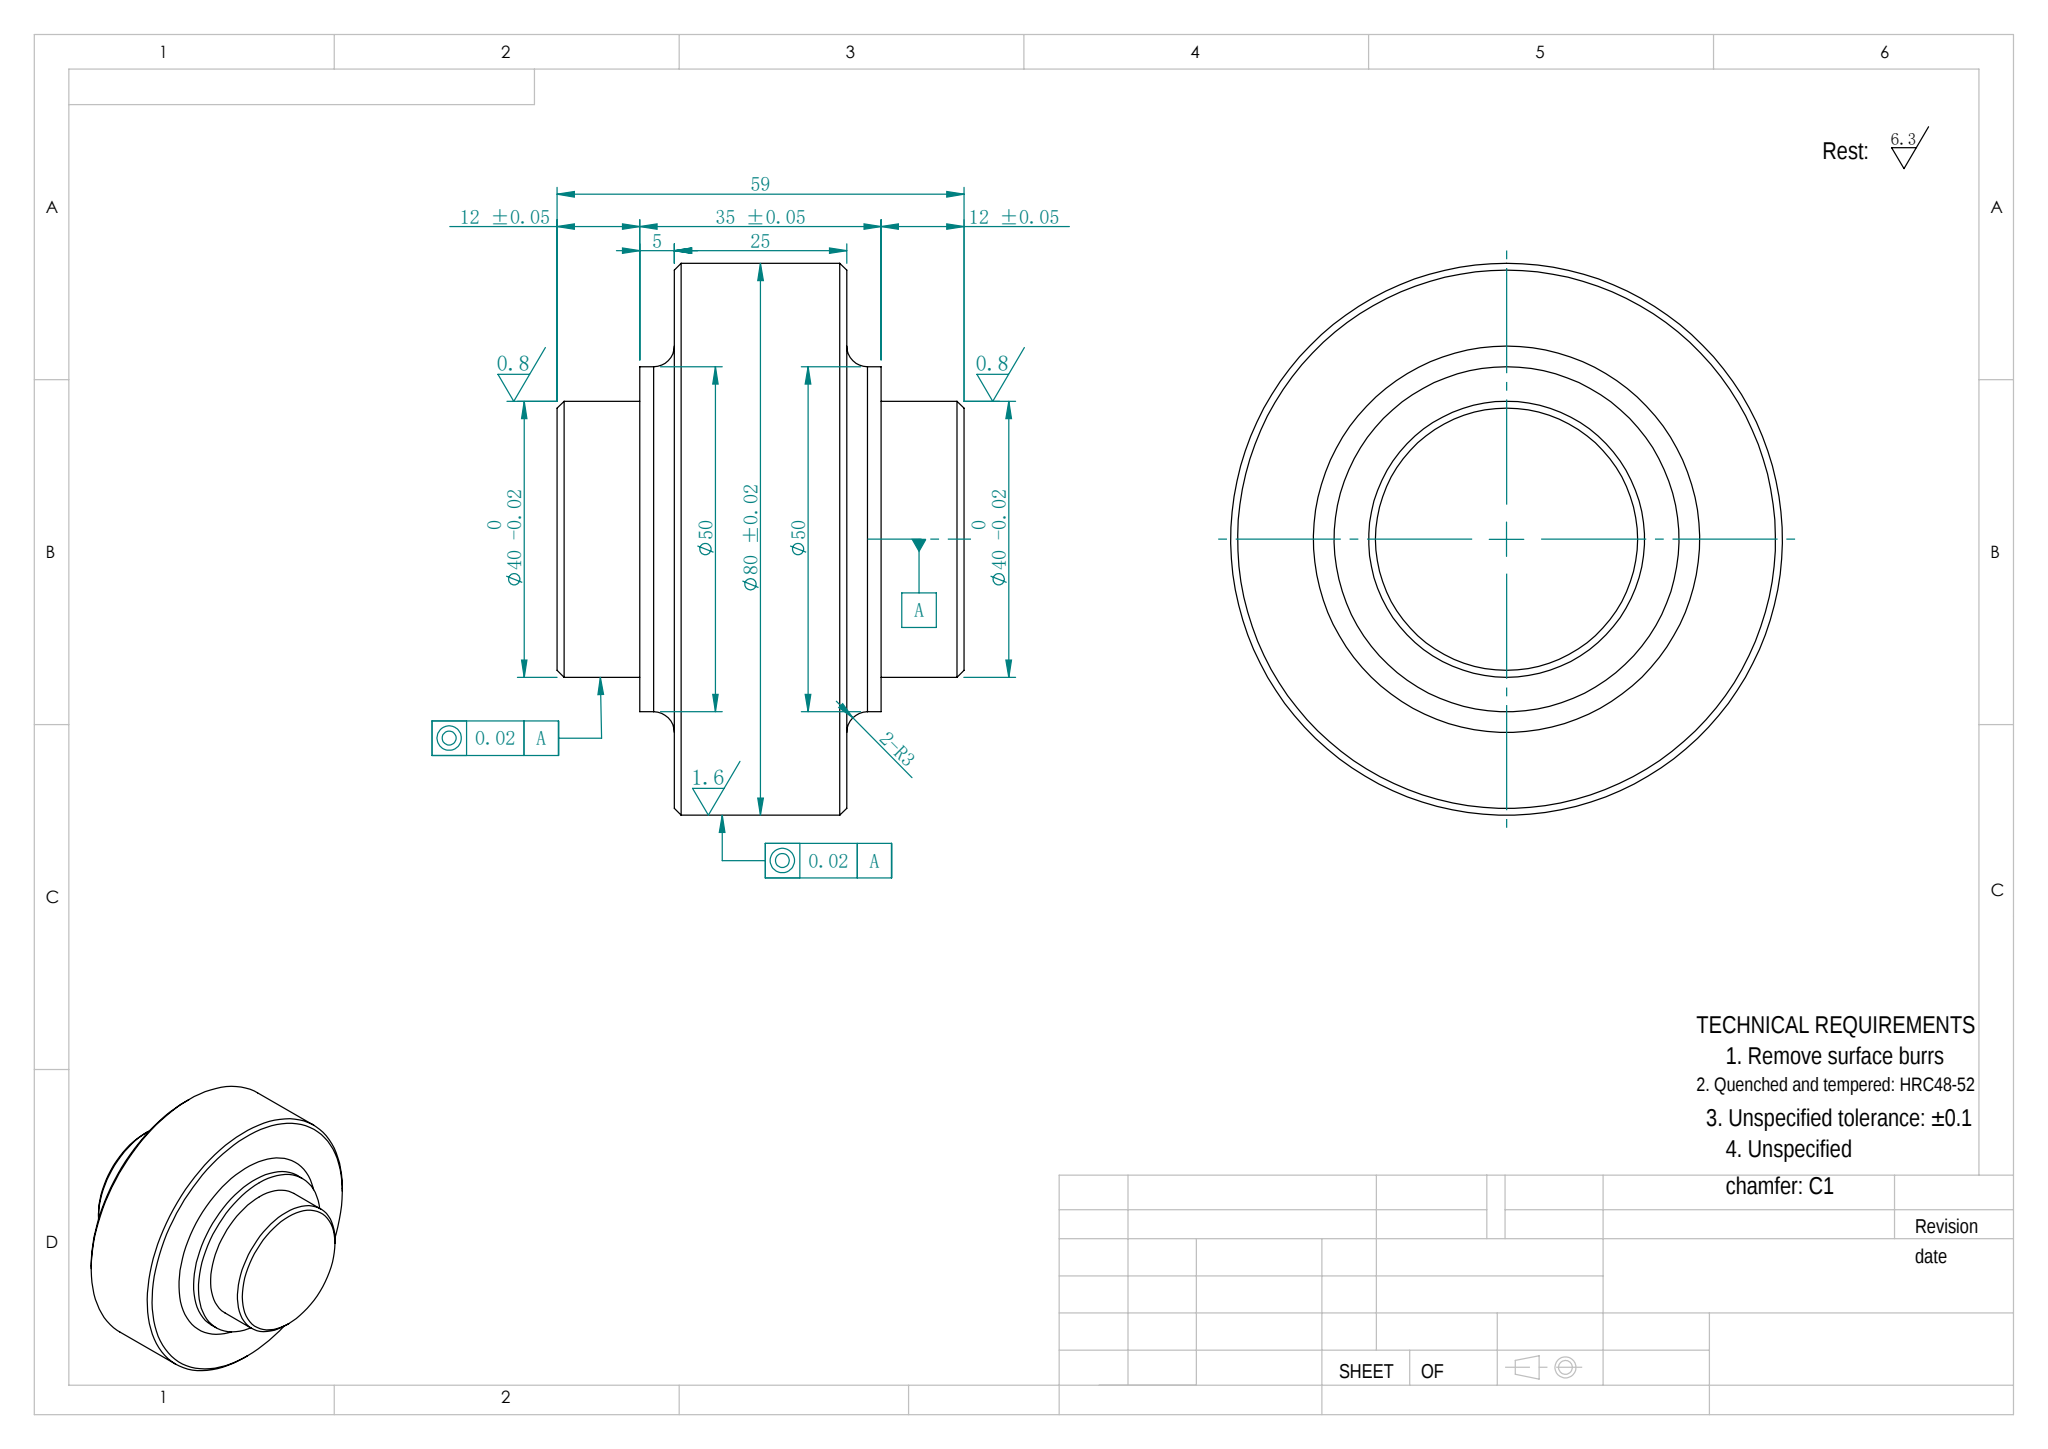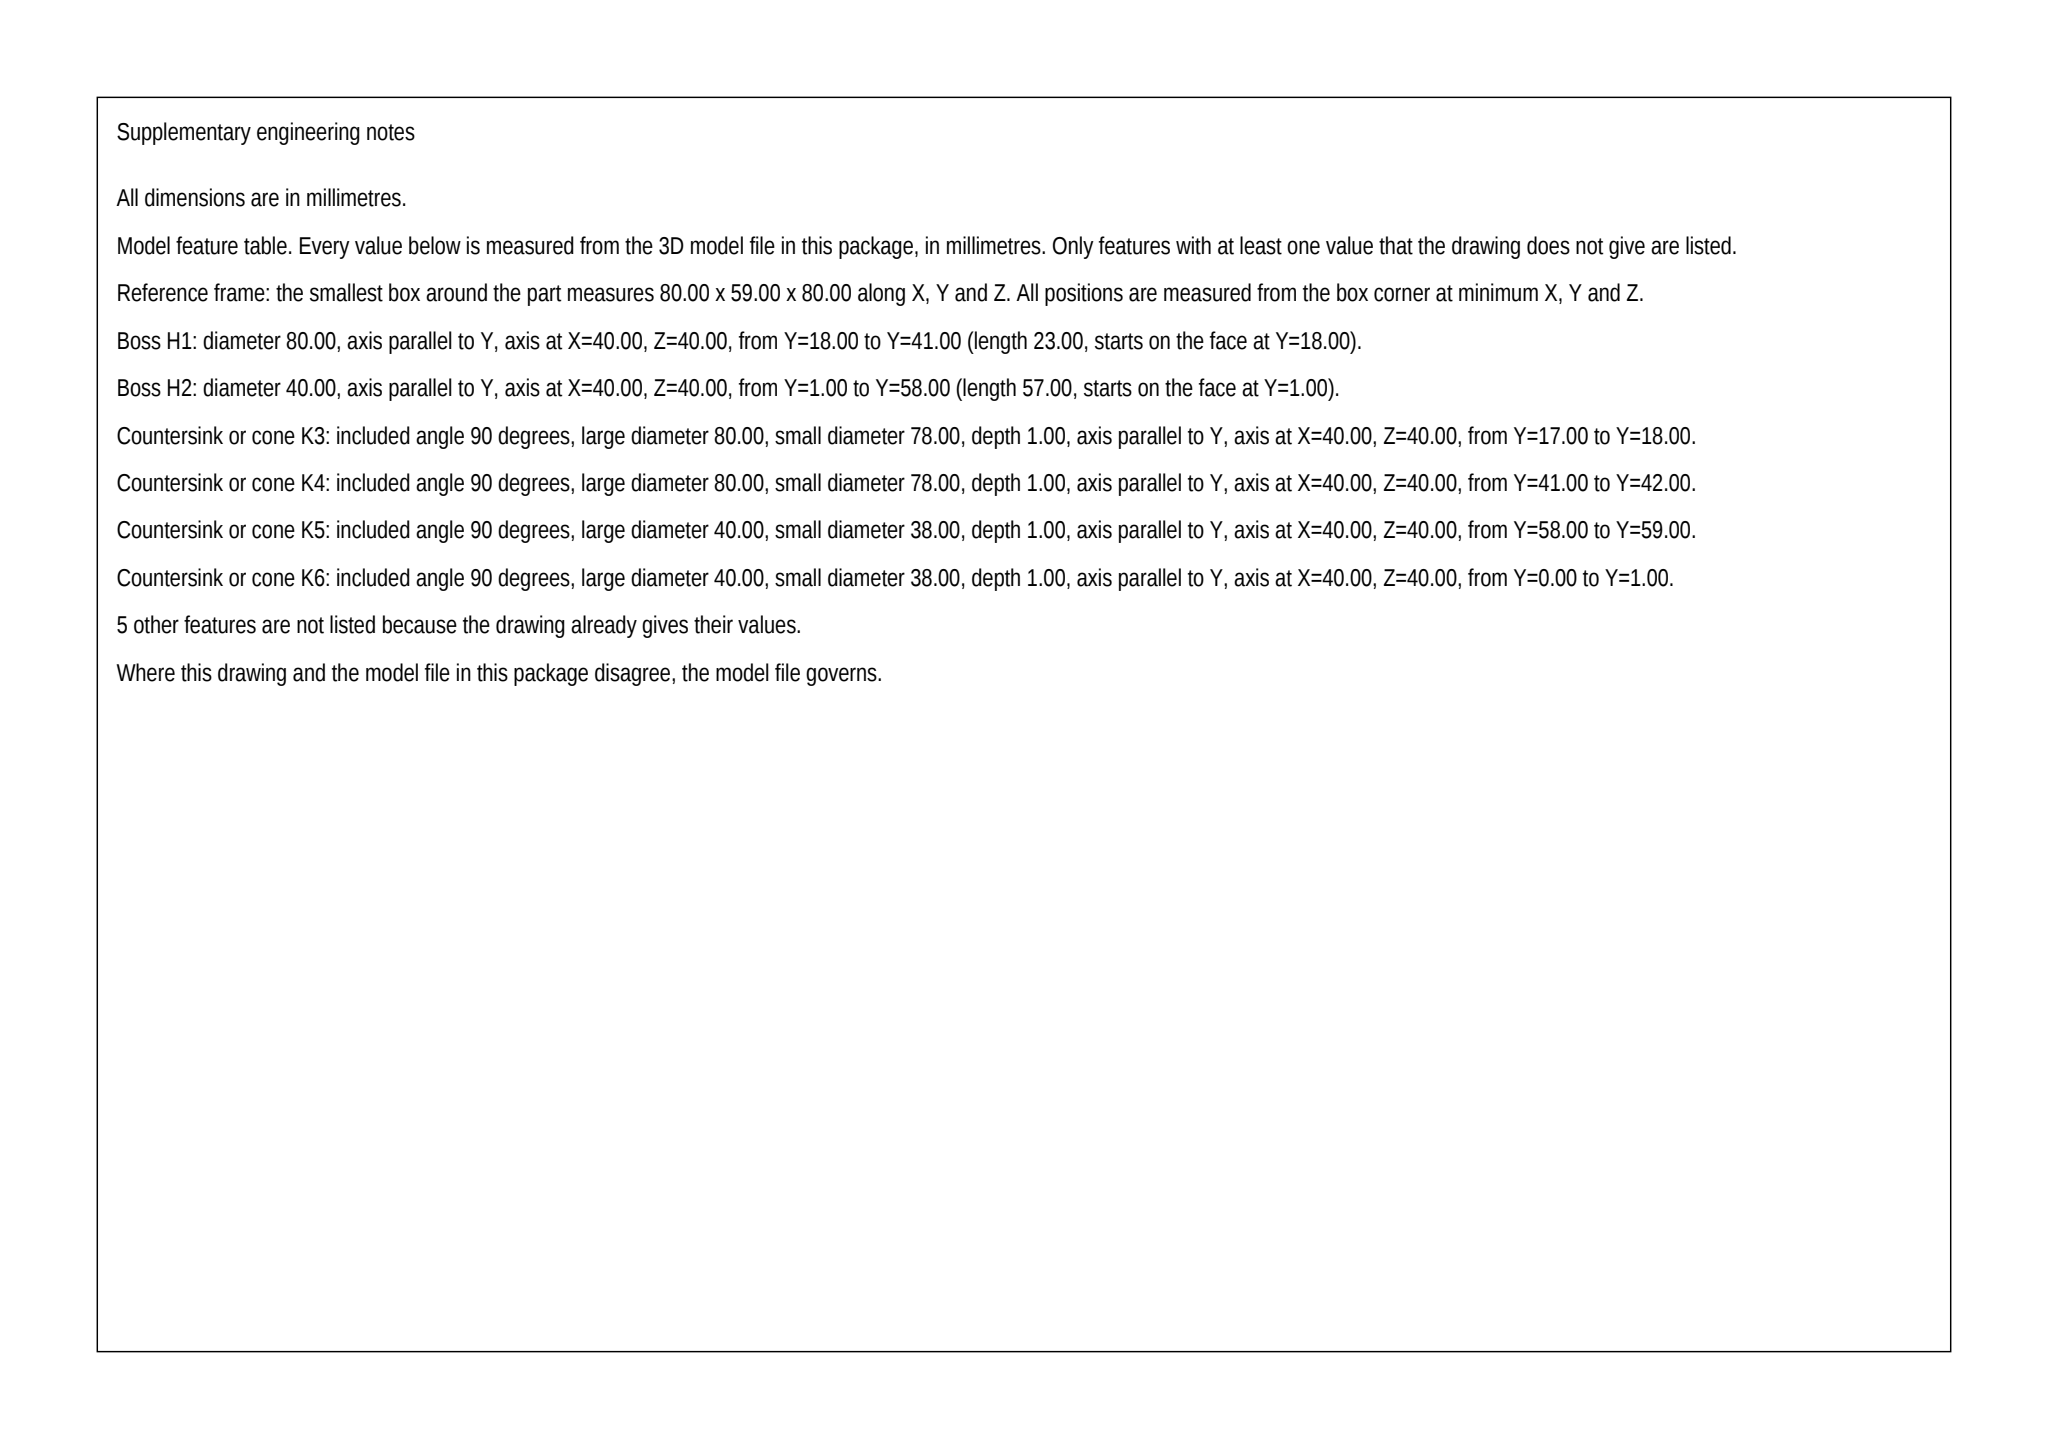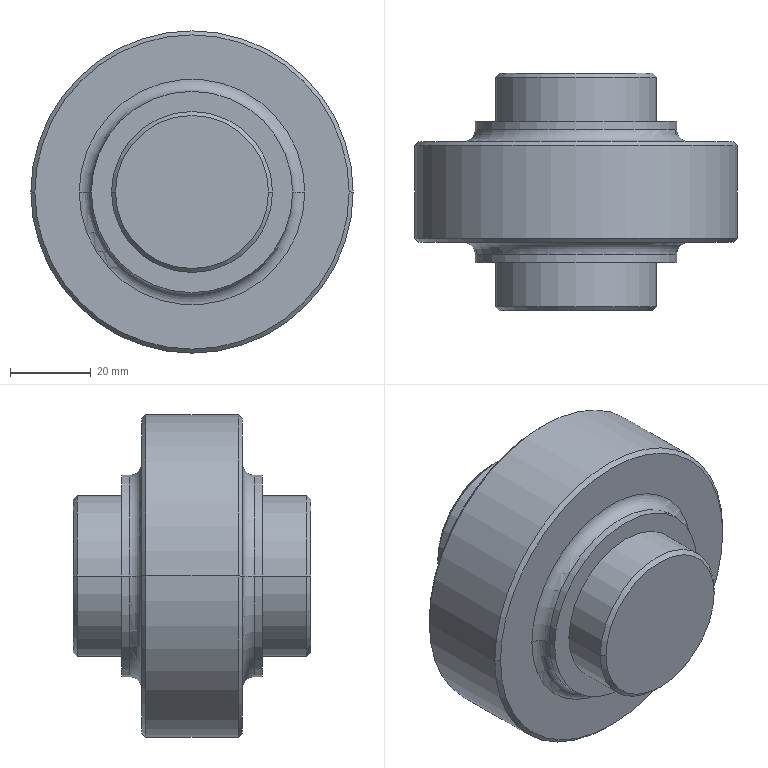Part | SolidWorks | mm | 1 solid | 28 faces | box 80 x 59 x 80 mm | volume 175708 mm3 | cylinder 10 | cone 8 | plane 6 | torus 4 | commonest cylinder face diameters 40 x4 50 x4 80 x2
build123d program:
from build123d import *

# Parameters (mm, degrees)
CHAMFER1_SIZE = 1
FILLET2_R     = 3


with BuildPart() as part:
    # Sketch1 → Revolve1 (revolve)
    with BuildSketch(Plane.XY, mode=Mode.PRIVATE) as revolve1_sk:
        Polygon((0, 59), (-20, 59), (-20, 47), (-25, 47), (-25, 42), (-40, 42), (-40, 17), (-25, 17), (-25, 12), (-20, 12), (-20, 0), (0, 0), align=None)
    revolve(revolve1_sk.sketch.rotate(Axis((0, 0, 0), (0, 1, 0)), 180), axis=Axis((0, 0, 0), (0, 1, 0)))

    # Chamfer1
    chamfer1_edges = [part.edges().sort_by_distance(p)[0] for p in [
        (-40, 17, 0),
        (-40, 42, 0),
        (-20, 59, 0),
        (-20, 0, 0),
    ]]
    chamfer(chamfer1_edges, length=CHAMFER1_SIZE)

    # Fillet2
    fillet2_edges = [part.edges().sort_by_distance(p)[0] for p in [
        (-25, 17, 0),
        (-25, 42, 0),
    ]]
    fillet(fillet2_edges, radius=FILLET2_R)


solid = part.part
STEP:
#1=CARTESIAN_POINT('',(28.,17.,0.));
#2=VERTEX_POINT('',#1);
#3=CARTESIAN_POINT('',(-28.,17.,0.));
#4=VERTEX_POINT('',#3);
#5=CARTESIAN_POINT('',(0.,17.,0.));
#6=DIRECTION('',(0.,1.,0.));
#7=DIRECTION('',(-1.,0.,0.));
#8=AXIS2_PLACEMENT_3D('',#5,#6,#7);
#9=CIRCLE('',#8,28.);
#10=EDGE_CURVE('',#2,#4,#9,.T.);
#11=ORIENTED_EDGE('',*,*,#10,.F.);
#12=CARTESIAN_POINT('',(25.,14.,0.));
#13=VERTEX_POINT('',#12);
#14=CARTESIAN_POINT('',(28.,14.,0.));
#15=DIRECTION('',(-0.,0.,1.));
#16=DIRECTION('',(1.,0.,0.));
#17=AXIS2_PLACEMENT_3D('',#14,#15,#16);
#18=CIRCLE('',#17,3.);
#19=EDGE_CURVE('',#2,#13,#18,.T.);
#20=ORIENTED_EDGE('',*,*,#19,.T.);
#21=CARTESIAN_POINT('',(-25.,14.,0.));
#22=VERTEX_POINT('',#21);
#23=CARTESIAN_POINT('',(0.,14.,0.));
#24=DIRECTION('',(-0.,-1.,0.));
#25=DIRECTION('',(-1.,0.,0.));
#26=AXIS2_PLACEMENT_3D('',#23,#24,#25);
#27=CIRCLE('',#26,25.);
#28=EDGE_CURVE('',#22,#13,#27,.T.);
#29=ORIENTED_EDGE('',*,*,#28,.F.);
#30=CARTESIAN_POINT('',(-28.,14.,0.));
#31=DIRECTION('',(0.,0.,-1.));
#32=DIRECTION('',(-1.,0.,0.));
#33=AXIS2_PLACEMENT_3D('',#30,#31,#32);
#34=CIRCLE('',#33,3.);
#35=EDGE_CURVE('',#4,#22,#34,.T.);
#36=ORIENTED_EDGE('',*,*,#35,.F.);
#37=EDGE_LOOP('',(#11,#20,#29,#36));
#38=FACE_OUTER_BOUND('',#37,.T.);
#39=CARTESIAN_POINT('',(0.,14.,0.));
#40=DIRECTION('',(0.,1.,0.));
#41=DIRECTION('',(-1.,0.,0.));
#42=AXIS2_PLACEMENT_3D('',#39,#40,#41);
#43=TOROIDAL_SURFACE('',#42,28.,3.);
#44=ADVANCED_FACE('',(#38),#43,.F.);
#45=CARTESIAN_POINT('',(-28.,42.,0.));
#46=VERTEX_POINT('',#45);
#47=CARTESIAN_POINT('',(28.,42.,0.));
#48=VERTEX_POINT('',#47);
#49=CARTESIAN_POINT('',(0.,42.,0.));
#50=DIRECTION('',(-0.,-1.,0.));
#51=DIRECTION('',(1.,0.,0.));
#52=AXIS2_PLACEMENT_3D('',#49,#50,#51);
#53=CIRCLE('',#52,28.);
#54=EDGE_CURVE('',#46,#48,#53,.T.);
#55=ORIENTED_EDGE('',*,*,#54,.F.);
#56=CARTESIAN_POINT('',(-25.,45.,0.));
#57=VERTEX_POINT('',#56);
#58=CARTESIAN_POINT('',(-28.,45.,0.));
#59=DIRECTION('',(0.,-0.,1.));
#60=DIRECTION('',(1.,0.,-0.));
#61=AXIS2_PLACEMENT_3D('',#58,#59,#60);
#62=CIRCLE('',#61,3.);
#63=EDGE_CURVE('',#46,#57,#62,.T.);
#64=ORIENTED_EDGE('',*,*,#63,.T.);
#65=CARTESIAN_POINT('',(25.,45.,0.));
#66=VERTEX_POINT('',#65);
#67=CARTESIAN_POINT('',(0.,45.,0.));
#68=DIRECTION('',(0.,1.,0.));
#69=DIRECTION('',(1.,0.,0.));
#70=AXIS2_PLACEMENT_3D('',#67,#68,#69);
#71=CIRCLE('',#70,25.);
#72=EDGE_CURVE('',#66,#57,#71,.T.);
#73=ORIENTED_EDGE('',*,*,#72,.F.);
#74=CARTESIAN_POINT('',(28.,45.,0.));
#75=DIRECTION('',(0.,0.,-1.));
#76=DIRECTION('',(-1.,0.,0.));
#77=AXIS2_PLACEMENT_3D('',#74,#75,#76);
#78=CIRCLE('',#77,3.);
#79=EDGE_CURVE('',#48,#66,#78,.T.);
#80=ORIENTED_EDGE('',*,*,#79,.F.);
#81=EDGE_LOOP('',(#55,#64,#73,#80));
#82=FACE_OUTER_BOUND('',#81,.T.);
#83=CARTESIAN_POINT('',(0.,45.,0.));
#84=DIRECTION('',(-0.,-1.,0.));
#85=DIRECTION('',(1.,-0.,0.));
#86=AXIS2_PLACEMENT_3D('',#83,#84,#85);
#87=TOROIDAL_SURFACE('',#86,28.,3.);
#88=ADVANCED_FACE('',(#82),#87,.F.);
#89=CARTESIAN_POINT('',(19.,-0.,0.));
#90=VERTEX_POINT('',#89);
#91=CARTESIAN_POINT('',(-19.,0.,0.));
#92=VERTEX_POINT('',#91);
#93=CARTESIAN_POINT('',(-0.,-0.,0.));
#94=DIRECTION('',(-0.,-1.,0.));
#95=DIRECTION('',(-1.,0.,0.));
#96=AXIS2_PLACEMENT_3D('',#93,#94,#95);
#97=CIRCLE('',#96,19.);
#98=EDGE_CURVE('',#90,#92,#97,.T.);
#99=ORIENTED_EDGE('',*,*,#98,.F.);
#100=CARTESIAN_POINT('',(20.,1.,0.));
#101=VERTEX_POINT('',#100);
#102=CARTESIAN_POINT('',(19.,-0.,0.));
#103=DIRECTION('',(0.7071,0.7071,0.));
#104=VECTOR('',#103,1000.);
#105=LINE('',#102,#104);
#106=EDGE_CURVE('',#90,#101,#105,.T.);
#107=ORIENTED_EDGE('',*,*,#106,.T.);
#108=CARTESIAN_POINT('',(-20.,1.,0.));
#109=VERTEX_POINT('',#108);
#110=CARTESIAN_POINT('',(0.,1.,0.));
#111=DIRECTION('',(0.,1.,0.));
#112=DIRECTION('',(-1.,0.,0.));
#113=AXIS2_PLACEMENT_3D('',#110,#111,#112);
#114=CIRCLE('',#113,20.);
#115=EDGE_CURVE('',#109,#101,#114,.T.);
#116=ORIENTED_EDGE('',*,*,#115,.F.);
#117=CARTESIAN_POINT('',(-19.,0.,0.));
#118=DIRECTION('',(-0.7071,0.7071,0.));
#119=VECTOR('',#118,1000.);
#120=LINE('',#117,#119);
#121=EDGE_CURVE('',#92,#109,#120,.T.);
#122=ORIENTED_EDGE('',*,*,#121,.F.);
#123=EDGE_LOOP('',(#99,#107,#116,#122));
#124=FACE_OUTER_BOUND('',#123,.T.);
#125=CARTESIAN_POINT('',(-0.,-0.,0.));
#126=DIRECTION('',(0.,1.,0.));
#127=DIRECTION('',(-1.,0.,0.));
#128=AXIS2_PLACEMENT_3D('',#125,#126,#127);
#129=CONICAL_SURFACE('',#128,19.,0.7854);
#130=ADVANCED_FACE('',(#124),#129,.T.);
#131=CARTESIAN_POINT('',(39.,17.,0.));
#132=VERTEX_POINT('',#131);
#133=CARTESIAN_POINT('',(-39.,17.,0.));
#134=VERTEX_POINT('',#133);
#135=CARTESIAN_POINT('',(0.,17.,0.));
#136=DIRECTION('',(-0.,-1.,0.));
#137=DIRECTION('',(-1.,0.,0.));
#138=AXIS2_PLACEMENT_3D('',#135,#136,#137);
#139=CIRCLE('',#138,39.);
#140=EDGE_CURVE('',#132,#134,#139,.T.);
#141=ORIENTED_EDGE('',*,*,#140,.F.);
#142=CARTESIAN_POINT('',(40.,18.,0.));
#143=VERTEX_POINT('',#142);
#144=CARTESIAN_POINT('',(39.,17.,0.));
#145=DIRECTION('',(0.7071,0.7071,0.));
#146=VECTOR('',#145,1000.);
#147=LINE('',#144,#146);
#148=EDGE_CURVE('',#132,#143,#147,.T.);
#149=ORIENTED_EDGE('',*,*,#148,.T.);
#150=CARTESIAN_POINT('',(-40.,18.,0.));
#151=VERTEX_POINT('',#150);
#152=CARTESIAN_POINT('',(0.,18.,0.));
#153=DIRECTION('',(0.,1.,0.));
#154=DIRECTION('',(-1.,0.,0.));
#155=AXIS2_PLACEMENT_3D('',#152,#153,#154);
#156=CIRCLE('',#155,40.);
#157=EDGE_CURVE('',#151,#143,#156,.T.);
#158=ORIENTED_EDGE('',*,*,#157,.F.);
#159=CARTESIAN_POINT('',(-39.,17.,0.));
#160=DIRECTION('',(-0.7071,0.7071,0.));
#161=VECTOR('',#160,1000.);
#162=LINE('',#159,#161);
#163=EDGE_CURVE('',#134,#151,#162,.T.);
#164=ORIENTED_EDGE('',*,*,#163,.F.);
#165=EDGE_LOOP('',(#141,#149,#158,#164));
#166=FACE_OUTER_BOUND('',#165,.T.);
#167=CARTESIAN_POINT('',(0.,17.,0.));
#168=DIRECTION('',(0.,1.,0.));
#169=DIRECTION('',(-1.,0.,0.));
#170=AXIS2_PLACEMENT_3D('',#167,#168,#169);
#171=CONICAL_SURFACE('',#170,39.,0.7854);
#172=ADVANCED_FACE('',(#166),#171,.T.);
#173=CARTESIAN_POINT('',(-39.,42.,0.));
#174=VERTEX_POINT('',#173);
#175=CARTESIAN_POINT('',(39.,42.,0.));
#176=VERTEX_POINT('',#175);
#177=CARTESIAN_POINT('',(0.,42.,0.));
#178=DIRECTION('',(0.,1.,0.));
#179=DIRECTION('',(1.,0.,0.));
#180=AXIS2_PLACEMENT_3D('',#177,#178,#179);
#181=CIRCLE('',#180,39.);
#182=EDGE_CURVE('',#174,#176,#181,.T.);
#183=ORIENTED_EDGE('',*,*,#182,.F.);
#184=CARTESIAN_POINT('',(-40.,41.,0.));
#185=VERTEX_POINT('',#184);
#186=CARTESIAN_POINT('',(-40.,41.,0.));
#187=DIRECTION('',(-0.7071,-0.7071,0.));
#188=VECTOR('',#187,1000.);
#189=LINE('',#186,#188);
#190=EDGE_CURVE('',#174,#185,#189,.T.);
#191=ORIENTED_EDGE('',*,*,#190,.T.);
#192=CARTESIAN_POINT('',(40.,41.,0.));
#193=VERTEX_POINT('',#192);
#194=CARTESIAN_POINT('',(0.,41.,0.));
#195=DIRECTION('',(-0.,-1.,0.));
#196=DIRECTION('',(1.,0.,0.));
#197=AXIS2_PLACEMENT_3D('',#194,#195,#196);
#198=CIRCLE('',#197,40.);
#199=EDGE_CURVE('',#193,#185,#198,.T.);
#200=ORIENTED_EDGE('',*,*,#199,.F.);
#201=CARTESIAN_POINT('',(40.,41.,0.));
#202=DIRECTION('',(0.7071,-0.7071,0.));
#203=VECTOR('',#202,1000.);
#204=LINE('',#201,#203);
#205=EDGE_CURVE('',#176,#193,#204,.T.);
#206=ORIENTED_EDGE('',*,*,#205,.F.);
#207=EDGE_LOOP('',(#183,#191,#200,#206));
#208=FACE_OUTER_BOUND('',#207,.T.);
#209=CARTESIAN_POINT('',(0.,41.,0.));
#210=DIRECTION('',(-0.,-1.,0.));
#211=DIRECTION('',(1.,0.,0.));
#212=AXIS2_PLACEMENT_3D('',#209,#210,#211);
#213=CONICAL_SURFACE('',#212,40.,0.7854);
#214=ADVANCED_FACE('',(#208),#213,.T.);
#215=CARTESIAN_POINT('',(-19.,59.,0.));
#216=VERTEX_POINT('',#215);
#217=CARTESIAN_POINT('',(19.,59.,0.));
#218=VERTEX_POINT('',#217);
#219=CARTESIAN_POINT('',(0.,59.,0.));
#220=DIRECTION('',(0.,1.,0.));
#221=DIRECTION('',(1.,0.,0.));
#222=AXIS2_PLACEMENT_3D('',#219,#220,#221);
#223=CIRCLE('',#222,19.);
#224=EDGE_CURVE('',#216,#218,#223,.T.);
#225=ORIENTED_EDGE('',*,*,#224,.F.);
#226=CARTESIAN_POINT('',(-20.,58.,0.));
#227=VERTEX_POINT('',#226);
#228=CARTESIAN_POINT('',(-20.,58.,0.));
#229=DIRECTION('',(-0.7071,-0.7071,0.));
#230=VECTOR('',#229,1000.);
#231=LINE('',#228,#230);
#232=EDGE_CURVE('',#216,#227,#231,.T.);
#233=ORIENTED_EDGE('',*,*,#232,.T.);
#234=CARTESIAN_POINT('',(20.,58.,0.));
#235=VERTEX_POINT('',#234);
#236=CARTESIAN_POINT('',(0.,58.,0.));
#237=DIRECTION('',(-0.,-1.,0.));
#238=DIRECTION('',(1.,0.,0.));
#239=AXIS2_PLACEMENT_3D('',#236,#237,#238);
#240=CIRCLE('',#239,20.);
#241=EDGE_CURVE('',#235,#227,#240,.T.);
#242=ORIENTED_EDGE('',*,*,#241,.F.);
#243=CARTESIAN_POINT('',(20.,58.,0.));
#244=DIRECTION('',(0.7071,-0.7071,0.));
#245=VECTOR('',#244,1000.);
#246=LINE('',#243,#245);
#247=EDGE_CURVE('',#218,#235,#246,.T.);
#248=ORIENTED_EDGE('',*,*,#247,.F.);
#249=EDGE_LOOP('',(#225,#233,#242,#248));
#250=FACE_OUTER_BOUND('',#249,.T.);
#251=CARTESIAN_POINT('',(0.,58.,0.));
#252=DIRECTION('',(-0.,-1.,0.));
#253=DIRECTION('',(1.,0.,0.));
#254=AXIS2_PLACEMENT_3D('',#251,#252,#253);
#255=CONICAL_SURFACE('',#254,20.,0.7854);
#256=ADVANCED_FACE('',(#250),#255,.T.);
#257=CARTESIAN_POINT('',(20.,12.,0.));
#258=VERTEX_POINT('',#257);
#259=CARTESIAN_POINT('',(-20.,12.,0.));
#260=VERTEX_POINT('',#259);
#261=CARTESIAN_POINT('',(0.,12.,0.));
#262=DIRECTION('',(-0.,-1.,0.));
#263=DIRECTION('',(1.,0.,0.));
#264=AXIS2_PLACEMENT_3D('',#261,#262,#263);
#265=CIRCLE('',#264,20.);
#266=EDGE_CURVE('',#258,#260,#265,.T.);
#267=ORIENTED_EDGE('',*,*,#266,.T.);
#268=CARTESIAN_POINT('',(-20.,0.,0.));
#269=DIRECTION('',(-0.,-1.,0.));
#270=VECTOR('',#269,1000.);
#271=LINE('',#268,#270);
#272=EDGE_CURVE('',#260,#109,#271,.T.);
#273=ORIENTED_EDGE('',*,*,#272,.T.);
#274=ORIENTED_EDGE('',*,*,#115,.T.);
#275=CARTESIAN_POINT('',(20.,-0.,0.));
#276=DIRECTION('',(-0.,-1.,0.));
#277=VECTOR('',#276,1000.);
#278=LINE('',#275,#277);
#279=EDGE_CURVE('',#258,#101,#278,.T.);
#280=ORIENTED_EDGE('',*,*,#279,.F.);
#281=EDGE_LOOP('',(#267,#273,#274,#280));
#282=FACE_OUTER_BOUND('',#281,.T.);
#283=CARTESIAN_POINT('',(0.,0.,0.));
#284=DIRECTION('',(-0.,-1.,0.));
#285=DIRECTION('',(1.,-0.,0.));
#286=AXIS2_PLACEMENT_3D('',#283,#284,#285);
#287=CYLINDRICAL_SURFACE('',#286,20.);
#288=ADVANCED_FACE('',(#282),#287,.T.);
#289=CARTESIAN_POINT('',(0.,14.,0.));
#290=DIRECTION('',(-0.,-1.,0.));
#291=DIRECTION('',(-1.,0.,0.));
#292=AXIS2_PLACEMENT_3D('',#289,#290,#291);
#293=CIRCLE('',#292,25.);
#294=EDGE_CURVE('',#13,#22,#293,.T.);
#295=ORIENTED_EDGE('',*,*,#294,.T.);
#296=CARTESIAN_POINT('',(-25.,12.,0.));
#297=VERTEX_POINT('',#296);
#298=CARTESIAN_POINT('',(-25.,0.,0.));
#299=DIRECTION('',(-0.,-1.,0.));
#300=VECTOR('',#299,1000.);
#301=LINE('',#298,#300);
#302=EDGE_CURVE('',#22,#297,#301,.T.);
#303=ORIENTED_EDGE('',*,*,#302,.T.);
#304=CARTESIAN_POINT('',(25.,12.,0.));
#305=VERTEX_POINT('',#304);
#306=CARTESIAN_POINT('',(0.,12.,0.));
#307=DIRECTION('',(-0.,-1.,0.));
#308=DIRECTION('',(1.,0.,0.));
#309=AXIS2_PLACEMENT_3D('',#306,#307,#308);
#310=CIRCLE('',#309,25.);
#311=EDGE_CURVE('',#305,#297,#310,.T.);
#312=ORIENTED_EDGE('',*,*,#311,.F.);
#313=CARTESIAN_POINT('',(25.,-0.,0.));
#314=DIRECTION('',(-0.,-1.,0.));
#315=VECTOR('',#314,1000.);
#316=LINE('',#313,#315);
#317=EDGE_CURVE('',#13,#305,#316,.T.);
#318=ORIENTED_EDGE('',*,*,#317,.F.);
#319=EDGE_LOOP('',(#295,#303,#312,#318));
#320=FACE_OUTER_BOUND('',#319,.T.);
#321=CARTESIAN_POINT('',(0.,0.,0.));
#322=DIRECTION('',(-0.,-1.,0.));
#323=DIRECTION('',(1.,-0.,0.));
#324=AXIS2_PLACEMENT_3D('',#321,#322,#323);
#325=CYLINDRICAL_SURFACE('',#324,25.);
#326=ADVANCED_FACE('',(#320),#325,.T.);
#327=ORIENTED_EDGE('',*,*,#199,.T.);
#328=CARTESIAN_POINT('',(-40.,0.,0.));
#329=DIRECTION('',(-0.,-1.,0.));
#330=VECTOR('',#329,1000.);
#331=LINE('',#328,#330);
#332=EDGE_CURVE('',#185,#151,#331,.T.);
#333=ORIENTED_EDGE('',*,*,#332,.T.);
#334=ORIENTED_EDGE('',*,*,#157,.T.);
#335=CARTESIAN_POINT('',(40.,-0.,0.));
#336=DIRECTION('',(-0.,-1.,0.));
#337=VECTOR('',#336,1000.);
#338=LINE('',#335,#337);
#339=EDGE_CURVE('',#193,#143,#338,.T.);
#340=ORIENTED_EDGE('',*,*,#339,.F.);
#341=EDGE_LOOP('',(#327,#333,#334,#340));
#342=FACE_OUTER_BOUND('',#341,.T.);
#343=CARTESIAN_POINT('',(0.,0.,0.));
#344=DIRECTION('',(-0.,-1.,0.));
#345=DIRECTION('',(1.,-0.,0.));
#346=AXIS2_PLACEMENT_3D('',#343,#344,#345);
#347=CYLINDRICAL_SURFACE('',#346,40.);
#348=ADVANCED_FACE('',(#342),#347,.T.);
#349=CARTESIAN_POINT('',(25.,47.,0.));
#350=VERTEX_POINT('',#349);
#351=CARTESIAN_POINT('',(-25.,47.,0.));
#352=VERTEX_POINT('',#351);
#353=CARTESIAN_POINT('',(0.,47.,0.));
#354=DIRECTION('',(-0.,-1.,0.));
#355=DIRECTION('',(1.,0.,0.));
#356=AXIS2_PLACEMENT_3D('',#353,#354,#355);
#357=CIRCLE('',#356,25.);
#358=EDGE_CURVE('',#350,#352,#357,.T.);
#359=ORIENTED_EDGE('',*,*,#358,.T.);
#360=CARTESIAN_POINT('',(-25.,0.,0.));
#361=DIRECTION('',(-0.,-1.,0.));
#362=VECTOR('',#361,1000.);
#363=LINE('',#360,#362);
#364=EDGE_CURVE('',#352,#57,#363,.T.);
#365=ORIENTED_EDGE('',*,*,#364,.T.);
#366=CARTESIAN_POINT('',(0.,45.,0.));
#367=DIRECTION('',(0.,1.,0.));
#368=DIRECTION('',(1.,0.,0.));
#369=AXIS2_PLACEMENT_3D('',#366,#367,#368);
#370=CIRCLE('',#369,25.);
#371=EDGE_CURVE('',#57,#66,#370,.T.);
#372=ORIENTED_EDGE('',*,*,#371,.T.);
#373=CARTESIAN_POINT('',(25.,-0.,0.));
#374=DIRECTION('',(-0.,-1.,0.));
#375=VECTOR('',#374,1000.);
#376=LINE('',#373,#375);
#377=EDGE_CURVE('',#350,#66,#376,.T.);
#378=ORIENTED_EDGE('',*,*,#377,.F.);
#379=EDGE_LOOP('',(#359,#365,#372,#378));
#380=FACE_OUTER_BOUND('',#379,.T.);
#381=CARTESIAN_POINT('',(0.,0.,0.));
#382=DIRECTION('',(-0.,-1.,0.));
#383=DIRECTION('',(1.,-0.,0.));
#384=AXIS2_PLACEMENT_3D('',#381,#382,#383);
#385=CYLINDRICAL_SURFACE('',#384,25.);
#386=ADVANCED_FACE('',(#380),#385,.T.);
#387=ORIENTED_EDGE('',*,*,#241,.T.);
#388=CARTESIAN_POINT('',(-20.,47.,0.));
#389=VERTEX_POINT('',#388);
#390=CARTESIAN_POINT('',(-20.,0.,0.));
#391=DIRECTION('',(-0.,-1.,0.));
#392=VECTOR('',#391,1000.);
#393=LINE('',#390,#392);
#394=EDGE_CURVE('',#227,#389,#393,.T.);
#395=ORIENTED_EDGE('',*,*,#394,.T.);
#396=CARTESIAN_POINT('',(20.,47.,0.));
#397=VERTEX_POINT('',#396);
#398=CARTESIAN_POINT('',(0.,47.,0.));
#399=DIRECTION('',(-0.,-1.,0.));
#400=DIRECTION('',(1.,0.,0.));
#401=AXIS2_PLACEMENT_3D('',#398,#399,#400);
#402=CIRCLE('',#401,20.);
#403=EDGE_CURVE('',#397,#389,#402,.T.);
#404=ORIENTED_EDGE('',*,*,#403,.F.);
#405=CARTESIAN_POINT('',(20.,-0.,0.));
#406=DIRECTION('',(-0.,-1.,0.));
#407=VECTOR('',#406,1000.);
#408=LINE('',#405,#407);
#409=EDGE_CURVE('',#235,#397,#408,.T.);
#410=ORIENTED_EDGE('',*,*,#409,.F.);
#411=EDGE_LOOP('',(#387,#395,#404,#410));
#412=FACE_OUTER_BOUND('',#411,.T.);
#413=CARTESIAN_POINT('',(0.,0.,0.));
#414=DIRECTION('',(-0.,-1.,0.));
#415=DIRECTION('',(1.,-0.,0.));
#416=AXIS2_PLACEMENT_3D('',#413,#414,#415);
#417=CYLINDRICAL_SURFACE('',#416,20.);
#418=ADVANCED_FACE('',(#412),#417,.T.);
#419=CARTESIAN_POINT('',(0.,59.,0.));
#420=DIRECTION('',(0.,1.,0.));
#421=DIRECTION('',(1.,0.,0.));
#422=AXIS2_PLACEMENT_3D('',#419,#420,#421);
#423=CIRCLE('',#422,19.);
#424=EDGE_CURVE('',#218,#216,#423,.T.);
#425=ORIENTED_EDGE('',*,*,#424,.T.);
#426=ORIENTED_EDGE('',*,*,#224,.T.);
#427=EDGE_LOOP('',(#425,#426));
#428=FACE_OUTER_BOUND('',#427,.T.);
#429=CARTESIAN_POINT('',(0.,59.,0.));
#430=DIRECTION('',(-0.,-1.,0.));
#431=DIRECTION('',(1.,-0.,0.));
#432=AXIS2_PLACEMENT_3D('',#429,#430,#431);
#433=PLANE('',#432);
#434=ADVANCED_FACE('',(#428),#433,.F.);
#435=ORIENTED_EDGE('',*,*,#394,.F.);
#436=CARTESIAN_POINT('',(0.,58.,0.));
#437=DIRECTION('',(-0.,-1.,0.));
#438=DIRECTION('',(1.,0.,0.));
#439=AXIS2_PLACEMENT_3D('',#436,#437,#438);
#440=CIRCLE('',#439,20.);
#441=EDGE_CURVE('',#227,#235,#440,.T.);
#442=ORIENTED_EDGE('',*,*,#441,.T.);
#443=ORIENTED_EDGE('',*,*,#409,.T.);
#444=CARTESIAN_POINT('',(0.,47.,0.));
#445=DIRECTION('',(-0.,-1.,0.));
#446=DIRECTION('',(1.,0.,0.));
#447=AXIS2_PLACEMENT_3D('',#444,#445,#446);
#448=CIRCLE('',#447,20.);
#449=EDGE_CURVE('',#389,#397,#448,.T.);
#450=ORIENTED_EDGE('',*,*,#449,.F.);
#451=EDGE_LOOP('',(#435,#442,#443,#450));
#452=FACE_OUTER_BOUND('',#451,.T.);
#453=CARTESIAN_POINT('',(0.,0.,0.));
#454=DIRECTION('',(-0.,-1.,0.));
#455=DIRECTION('',(1.,-0.,0.));
#456=AXIS2_PLACEMENT_3D('',#453,#454,#455);
#457=CYLINDRICAL_SURFACE('',#456,20.);
#458=ADVANCED_FACE('',(#452),#457,.T.);
#459=ORIENTED_EDGE('',*,*,#358,.F.);
#460=CARTESIAN_POINT('',(0.,47.,0.));
#461=DIRECTION('',(-0.,-1.,0.));
#462=DIRECTION('',(1.,0.,0.));
#463=AXIS2_PLACEMENT_3D('',#460,#461,#462);
#464=CIRCLE('',#463,25.);
#465=EDGE_CURVE('',#352,#350,#464,.T.);
#466=ORIENTED_EDGE('',*,*,#465,.F.);
#467=EDGE_LOOP('',(#459,#466));
#468=FACE_OUTER_BOUND('',#467,.T.);
#469=ORIENTED_EDGE('',*,*,#403,.T.);
#470=ORIENTED_EDGE('',*,*,#449,.T.);
#471=EDGE_LOOP('',(#469,#470));
#472=FACE_BOUND('',#471,.T.);
#473=CARTESIAN_POINT('',(-20.,47.,0.));
#474=DIRECTION('',(-0.,-1.,0.));
#475=DIRECTION('',(1.,-0.,0.));
#476=AXIS2_PLACEMENT_3D('',#473,#474,#475);
#477=PLANE('',#476);
#478=ADVANCED_FACE('',(#468,#472),#477,.F.);
#479=ORIENTED_EDGE('',*,*,#364,.F.);
#480=ORIENTED_EDGE('',*,*,#465,.T.);
#481=ORIENTED_EDGE('',*,*,#377,.T.);
#482=ORIENTED_EDGE('',*,*,#72,.T.);
#483=EDGE_LOOP('',(#479,#480,#481,#482));
#484=FACE_OUTER_BOUND('',#483,.T.);
#485=CARTESIAN_POINT('',(0.,0.,0.));
#486=DIRECTION('',(-0.,-1.,0.));
#487=DIRECTION('',(1.,-0.,0.));
#488=AXIS2_PLACEMENT_3D('',#485,#486,#487);
#489=CYLINDRICAL_SURFACE('',#488,25.);
#490=ADVANCED_FACE('',(#484),#489,.T.);
#491=CARTESIAN_POINT('',(0.,42.,0.));
#492=DIRECTION('',(-0.,-1.,0.));
#493=DIRECTION('',(1.,0.,0.));
#494=AXIS2_PLACEMENT_3D('',#491,#492,#493);
#495=CIRCLE('',#494,28.);
#496=EDGE_CURVE('',#48,#46,#495,.T.);
#497=ORIENTED_EDGE('',*,*,#496,.T.);
#498=ORIENTED_EDGE('',*,*,#54,.T.);
#499=EDGE_LOOP('',(#497,#498));
#500=FACE_BOUND('',#499,.T.);
#501=CARTESIAN_POINT('',(0.,42.,0.));
#502=DIRECTION('',(0.,1.,0.));
#503=DIRECTION('',(1.,0.,0.));
#504=AXIS2_PLACEMENT_3D('',#501,#502,#503);
#505=CIRCLE('',#504,39.);
#506=EDGE_CURVE('',#176,#174,#505,.T.);
#507=ORIENTED_EDGE('',*,*,#506,.T.);
#508=ORIENTED_EDGE('',*,*,#182,.T.);
#509=EDGE_LOOP('',(#507,#508));
#510=FACE_OUTER_BOUND('',#509,.T.);
#511=CARTESIAN_POINT('',(-25.,42.,0.));
#512=DIRECTION('',(-0.,-1.,0.));
#513=DIRECTION('',(1.,-0.,0.));
#514=AXIS2_PLACEMENT_3D('',#511,#512,#513);
#515=PLANE('',#514);
#516=ADVANCED_FACE('',(#500,#510),#515,.F.);
#517=ORIENTED_EDGE('',*,*,#332,.F.);
#518=CARTESIAN_POINT('',(0.,41.,0.));
#519=DIRECTION('',(-0.,-1.,0.));
#520=DIRECTION('',(1.,0.,0.));
#521=AXIS2_PLACEMENT_3D('',#518,#519,#520);
#522=CIRCLE('',#521,40.);
#523=EDGE_CURVE('',#185,#193,#522,.T.);
#524=ORIENTED_EDGE('',*,*,#523,.T.);
#525=ORIENTED_EDGE('',*,*,#339,.T.);
#526=CARTESIAN_POINT('',(0.,18.,0.));
#527=DIRECTION('',(0.,1.,0.));
#528=DIRECTION('',(-1.,0.,0.));
#529=AXIS2_PLACEMENT_3D('',#526,#527,#528);
#530=CIRCLE('',#529,40.);
#531=EDGE_CURVE('',#143,#151,#530,.T.);
#532=ORIENTED_EDGE('',*,*,#531,.T.);
#533=EDGE_LOOP('',(#517,#524,#525,#532));
#534=FACE_OUTER_BOUND('',#533,.T.);
#535=CARTESIAN_POINT('',(0.,0.,0.));
#536=DIRECTION('',(-0.,-1.,0.));
#537=DIRECTION('',(1.,-0.,0.));
#538=AXIS2_PLACEMENT_3D('',#535,#536,#537);
#539=CYLINDRICAL_SURFACE('',#538,40.);
#540=ADVANCED_FACE('',(#534),#539,.T.);
#541=CARTESIAN_POINT('',(0.,17.,0.));
#542=DIRECTION('',(0.,1.,0.));
#543=DIRECTION('',(-1.,0.,0.));
#544=AXIS2_PLACEMENT_3D('',#541,#542,#543);
#545=CIRCLE('',#544,28.);
#546=EDGE_CURVE('',#4,#2,#545,.T.);
#547=ORIENTED_EDGE('',*,*,#546,.T.);
#548=ORIENTED_EDGE('',*,*,#10,.T.);
#549=EDGE_LOOP('',(#547,#548));
#550=FACE_BOUND('',#549,.T.);
#551=CARTESIAN_POINT('',(0.,17.,0.));
#552=DIRECTION('',(-0.,-1.,0.));
#553=DIRECTION('',(-1.,0.,0.));
#554=AXIS2_PLACEMENT_3D('',#551,#552,#553);
#555=CIRCLE('',#554,39.);
#556=EDGE_CURVE('',#134,#132,#555,.T.);
#557=ORIENTED_EDGE('',*,*,#556,.T.);
#558=ORIENTED_EDGE('',*,*,#140,.T.);
#559=EDGE_LOOP('',(#557,#558));
#560=FACE_OUTER_BOUND('',#559,.T.);
#561=CARTESIAN_POINT('',(-40.,17.,0.));
#562=DIRECTION('',(0.,1.,0.));
#563=DIRECTION('',(-1.,0.,0.));
#564=AXIS2_PLACEMENT_3D('',#561,#562,#563);
#565=PLANE('',#564);
#566=ADVANCED_FACE('',(#550,#560),#565,.F.);
#567=ORIENTED_EDGE('',*,*,#302,.F.);
#568=ORIENTED_EDGE('',*,*,#28,.T.);
#569=ORIENTED_EDGE('',*,*,#317,.T.);
#570=CARTESIAN_POINT('',(0.,12.,0.));
#571=DIRECTION('',(-0.,-1.,0.));
#572=DIRECTION('',(1.,0.,0.));
#573=AXIS2_PLACEMENT_3D('',#570,#571,#572);
#574=CIRCLE('',#573,25.);
#575=EDGE_CURVE('',#297,#305,#574,.T.);
#576=ORIENTED_EDGE('',*,*,#575,.F.);
#577=EDGE_LOOP('',(#567,#568,#569,#576));
#578=FACE_OUTER_BOUND('',#577,.T.);
#579=CARTESIAN_POINT('',(0.,0.,0.));
#580=DIRECTION('',(-0.,-1.,0.));
#581=DIRECTION('',(1.,-0.,0.));
#582=AXIS2_PLACEMENT_3D('',#579,#580,#581);
#583=CYLINDRICAL_SURFACE('',#582,25.);
#584=ADVANCED_FACE('',(#578),#583,.T.);
#585=ORIENTED_EDGE('',*,*,#266,.F.);
#586=CARTESIAN_POINT('',(0.,12.,0.));
#587=DIRECTION('',(-0.,-1.,0.));
#588=DIRECTION('',(1.,0.,0.));
#589=AXIS2_PLACEMENT_3D('',#586,#587,#588);
#590=CIRCLE('',#589,20.);
#591=EDGE_CURVE('',#260,#258,#590,.T.);
#592=ORIENTED_EDGE('',*,*,#591,.F.);
#593=EDGE_LOOP('',(#585,#592));
#594=FACE_BOUND('',#593,.T.);
#595=ORIENTED_EDGE('',*,*,#311,.T.);
#596=ORIENTED_EDGE('',*,*,#575,.T.);
#597=EDGE_LOOP('',(#595,#596));
#598=FACE_OUTER_BOUND('',#597,.T.);
#599=CARTESIAN_POINT('',(-25.,12.,0.));
#600=DIRECTION('',(0.,1.,0.));
#601=DIRECTION('',(-1.,0.,0.));
#602=AXIS2_PLACEMENT_3D('',#599,#600,#601);
#603=PLANE('',#602);
#604=ADVANCED_FACE('',(#594,#598),#603,.F.);
#605=ORIENTED_EDGE('',*,*,#272,.F.);
#606=ORIENTED_EDGE('',*,*,#591,.T.);
#607=ORIENTED_EDGE('',*,*,#279,.T.);
#608=CARTESIAN_POINT('',(0.,1.,0.));
#609=DIRECTION('',(0.,1.,0.));
#610=DIRECTION('',(-1.,0.,0.));
#611=AXIS2_PLACEMENT_3D('',#608,#609,#610);
#612=CIRCLE('',#611,20.);
#613=EDGE_CURVE('',#101,#109,#612,.T.);
#614=ORIENTED_EDGE('',*,*,#613,.T.);
#615=EDGE_LOOP('',(#605,#606,#607,#614));
#616=FACE_OUTER_BOUND('',#615,.T.);
#617=CARTESIAN_POINT('',(0.,0.,0.));
#618=DIRECTION('',(-0.,-1.,0.));
#619=DIRECTION('',(1.,-0.,0.));
#620=AXIS2_PLACEMENT_3D('',#617,#618,#619);
#621=CYLINDRICAL_SURFACE('',#620,20.);
#622=ADVANCED_FACE('',(#616),#621,.T.);
#623=CARTESIAN_POINT('',(-0.,-0.,0.));
#624=DIRECTION('',(-0.,-1.,0.));
#625=DIRECTION('',(-1.,0.,0.));
#626=AXIS2_PLACEMENT_3D('',#623,#624,#625);
#627=CIRCLE('',#626,19.);
#628=EDGE_CURVE('',#92,#90,#627,.T.);
#629=ORIENTED_EDGE('',*,*,#628,.T.);
#630=ORIENTED_EDGE('',*,*,#98,.T.);
#631=EDGE_LOOP('',(#629,#630));
#632=FACE_OUTER_BOUND('',#631,.T.);
#633=CARTESIAN_POINT('',(-20.,0.,0.));
#634=DIRECTION('',(0.,1.,0.));
#635=DIRECTION('',(-1.,0.,0.));
#636=AXIS2_PLACEMENT_3D('',#633,#634,#635);
#637=PLANE('',#636);
#638=ADVANCED_FACE('',(#632),#637,.F.);
#639=ORIENTED_EDGE('',*,*,#232,.F.);
#640=ORIENTED_EDGE('',*,*,#424,.F.);
#641=ORIENTED_EDGE('',*,*,#247,.T.);
#642=ORIENTED_EDGE('',*,*,#441,.F.);
#643=EDGE_LOOP('',(#639,#640,#641,#642));
#644=FACE_OUTER_BOUND('',#643,.T.);
#645=CARTESIAN_POINT('',(0.,58.,0.));
#646=DIRECTION('',(-0.,-1.,0.));
#647=DIRECTION('',(1.,0.,0.));
#648=AXIS2_PLACEMENT_3D('',#645,#646,#647);
#649=CONICAL_SURFACE('',#648,20.,0.7854);
#650=ADVANCED_FACE('',(#644),#649,.T.);
#651=ORIENTED_EDGE('',*,*,#190,.F.);
#652=ORIENTED_EDGE('',*,*,#506,.F.);
#653=ORIENTED_EDGE('',*,*,#205,.T.);
#654=ORIENTED_EDGE('',*,*,#523,.F.);
#655=EDGE_LOOP('',(#651,#652,#653,#654));
#656=FACE_OUTER_BOUND('',#655,.T.);
#657=CARTESIAN_POINT('',(0.,41.,0.));
#658=DIRECTION('',(-0.,-1.,0.));
#659=DIRECTION('',(1.,0.,0.));
#660=AXIS2_PLACEMENT_3D('',#657,#658,#659);
#661=CONICAL_SURFACE('',#660,40.,0.7854);
#662=ADVANCED_FACE('',(#656),#661,.T.);
#663=ORIENTED_EDGE('',*,*,#148,.F.);
#664=ORIENTED_EDGE('',*,*,#556,.F.);
#665=ORIENTED_EDGE('',*,*,#163,.T.);
#666=ORIENTED_EDGE('',*,*,#531,.F.);
#667=EDGE_LOOP('',(#663,#664,#665,#666));
#668=FACE_OUTER_BOUND('',#667,.T.);
#669=CARTESIAN_POINT('',(0.,17.,0.));
#670=DIRECTION('',(0.,1.,0.));
#671=DIRECTION('',(-1.,0.,0.));
#672=AXIS2_PLACEMENT_3D('',#669,#670,#671);
#673=CONICAL_SURFACE('',#672,39.,0.7854);
#674=ADVANCED_FACE('',(#668),#673,.T.);
#675=ORIENTED_EDGE('',*,*,#106,.F.);
#676=ORIENTED_EDGE('',*,*,#628,.F.);
#677=ORIENTED_EDGE('',*,*,#121,.T.);
#678=ORIENTED_EDGE('',*,*,#613,.F.);
#679=EDGE_LOOP('',(#675,#676,#677,#678));
#680=FACE_OUTER_BOUND('',#679,.T.);
#681=CARTESIAN_POINT('',(-0.,-0.,0.));
#682=DIRECTION('',(0.,1.,0.));
#683=DIRECTION('',(-1.,0.,0.));
#684=AXIS2_PLACEMENT_3D('',#681,#682,#683);
#685=CONICAL_SURFACE('',#684,19.,0.7854);
#686=ADVANCED_FACE('',(#680),#685,.T.);
#687=ORIENTED_EDGE('',*,*,#63,.F.);
#688=ORIENTED_EDGE('',*,*,#496,.F.);
#689=ORIENTED_EDGE('',*,*,#79,.T.);
#690=ORIENTED_EDGE('',*,*,#371,.F.);
#691=EDGE_LOOP('',(#687,#688,#689,#690));
#692=FACE_OUTER_BOUND('',#691,.T.);
#693=CARTESIAN_POINT('',(0.,45.,0.));
#694=DIRECTION('',(-0.,-1.,0.));
#695=DIRECTION('',(1.,-0.,0.));
#696=AXIS2_PLACEMENT_3D('',#693,#694,#695);
#697=TOROIDAL_SURFACE('',#696,28.,3.);
#698=ADVANCED_FACE('',(#692),#697,.F.);
#699=ORIENTED_EDGE('',*,*,#19,.F.);
#700=ORIENTED_EDGE('',*,*,#546,.F.);
#701=ORIENTED_EDGE('',*,*,#35,.T.);
#702=ORIENTED_EDGE('',*,*,#294,.F.);
#703=EDGE_LOOP('',(#699,#700,#701,#702));
#704=FACE_OUTER_BOUND('',#703,.T.);
#705=CARTESIAN_POINT('',(0.,14.,0.));
#706=DIRECTION('',(0.,1.,0.));
#707=DIRECTION('',(-1.,0.,0.));
#708=AXIS2_PLACEMENT_3D('',#705,#706,#707);
#709=TOROIDAL_SURFACE('',#708,28.,3.);
#710=ADVANCED_FACE('',(#704),#709,.F.);
#711=CLOSED_SHELL('',(#44,#88,#130,#172,#214,#256,#288,#326,#348,#386,#418,#434,#458,#478,#490,#516,#540,#566,#584,#604,#622,#638,#650,#662,#674,#686,#698,#710));
#712=MANIFOLD_SOLID_BREP('',#711);
#713=CARTESIAN_POINT('',(0.,0.,0.));
#714=DIRECTION('',(0.,0.,1.));
#715=DIRECTION('',(1.,0.,0.));
#716=AXIS2_PLACEMENT_3D('',#713,#714,#715);
#717=(LENGTH_UNIT()NAMED_UNIT(*)SI_UNIT(.MILLI.,.METRE.));
#718=UNCERTAINTY_MEASURE_WITH_UNIT(LENGTH_MEASURE(0.00001),#717,'','');
#719=(NAMED_UNIT(*)PLANE_ANGLE_UNIT()SI_UNIT($,.RADIAN.));
#720=(NAMED_UNIT(*)SI_UNIT($,.STERADIAN.)SOLID_ANGLE_UNIT());
#721=(GEOMETRIC_REPRESENTATION_CONTEXT(3)GLOBAL_UNCERTAINTY_ASSIGNED_CONTEXT((#718))GLOBAL_UNIT_ASSIGNED_CONTEXT((#717,#719,#720))REPRESENTATION_CONTEXT('',''));
#722=ADVANCED_BREP_SHAPE_REPRESENTATION('',(#712,#716),#721);